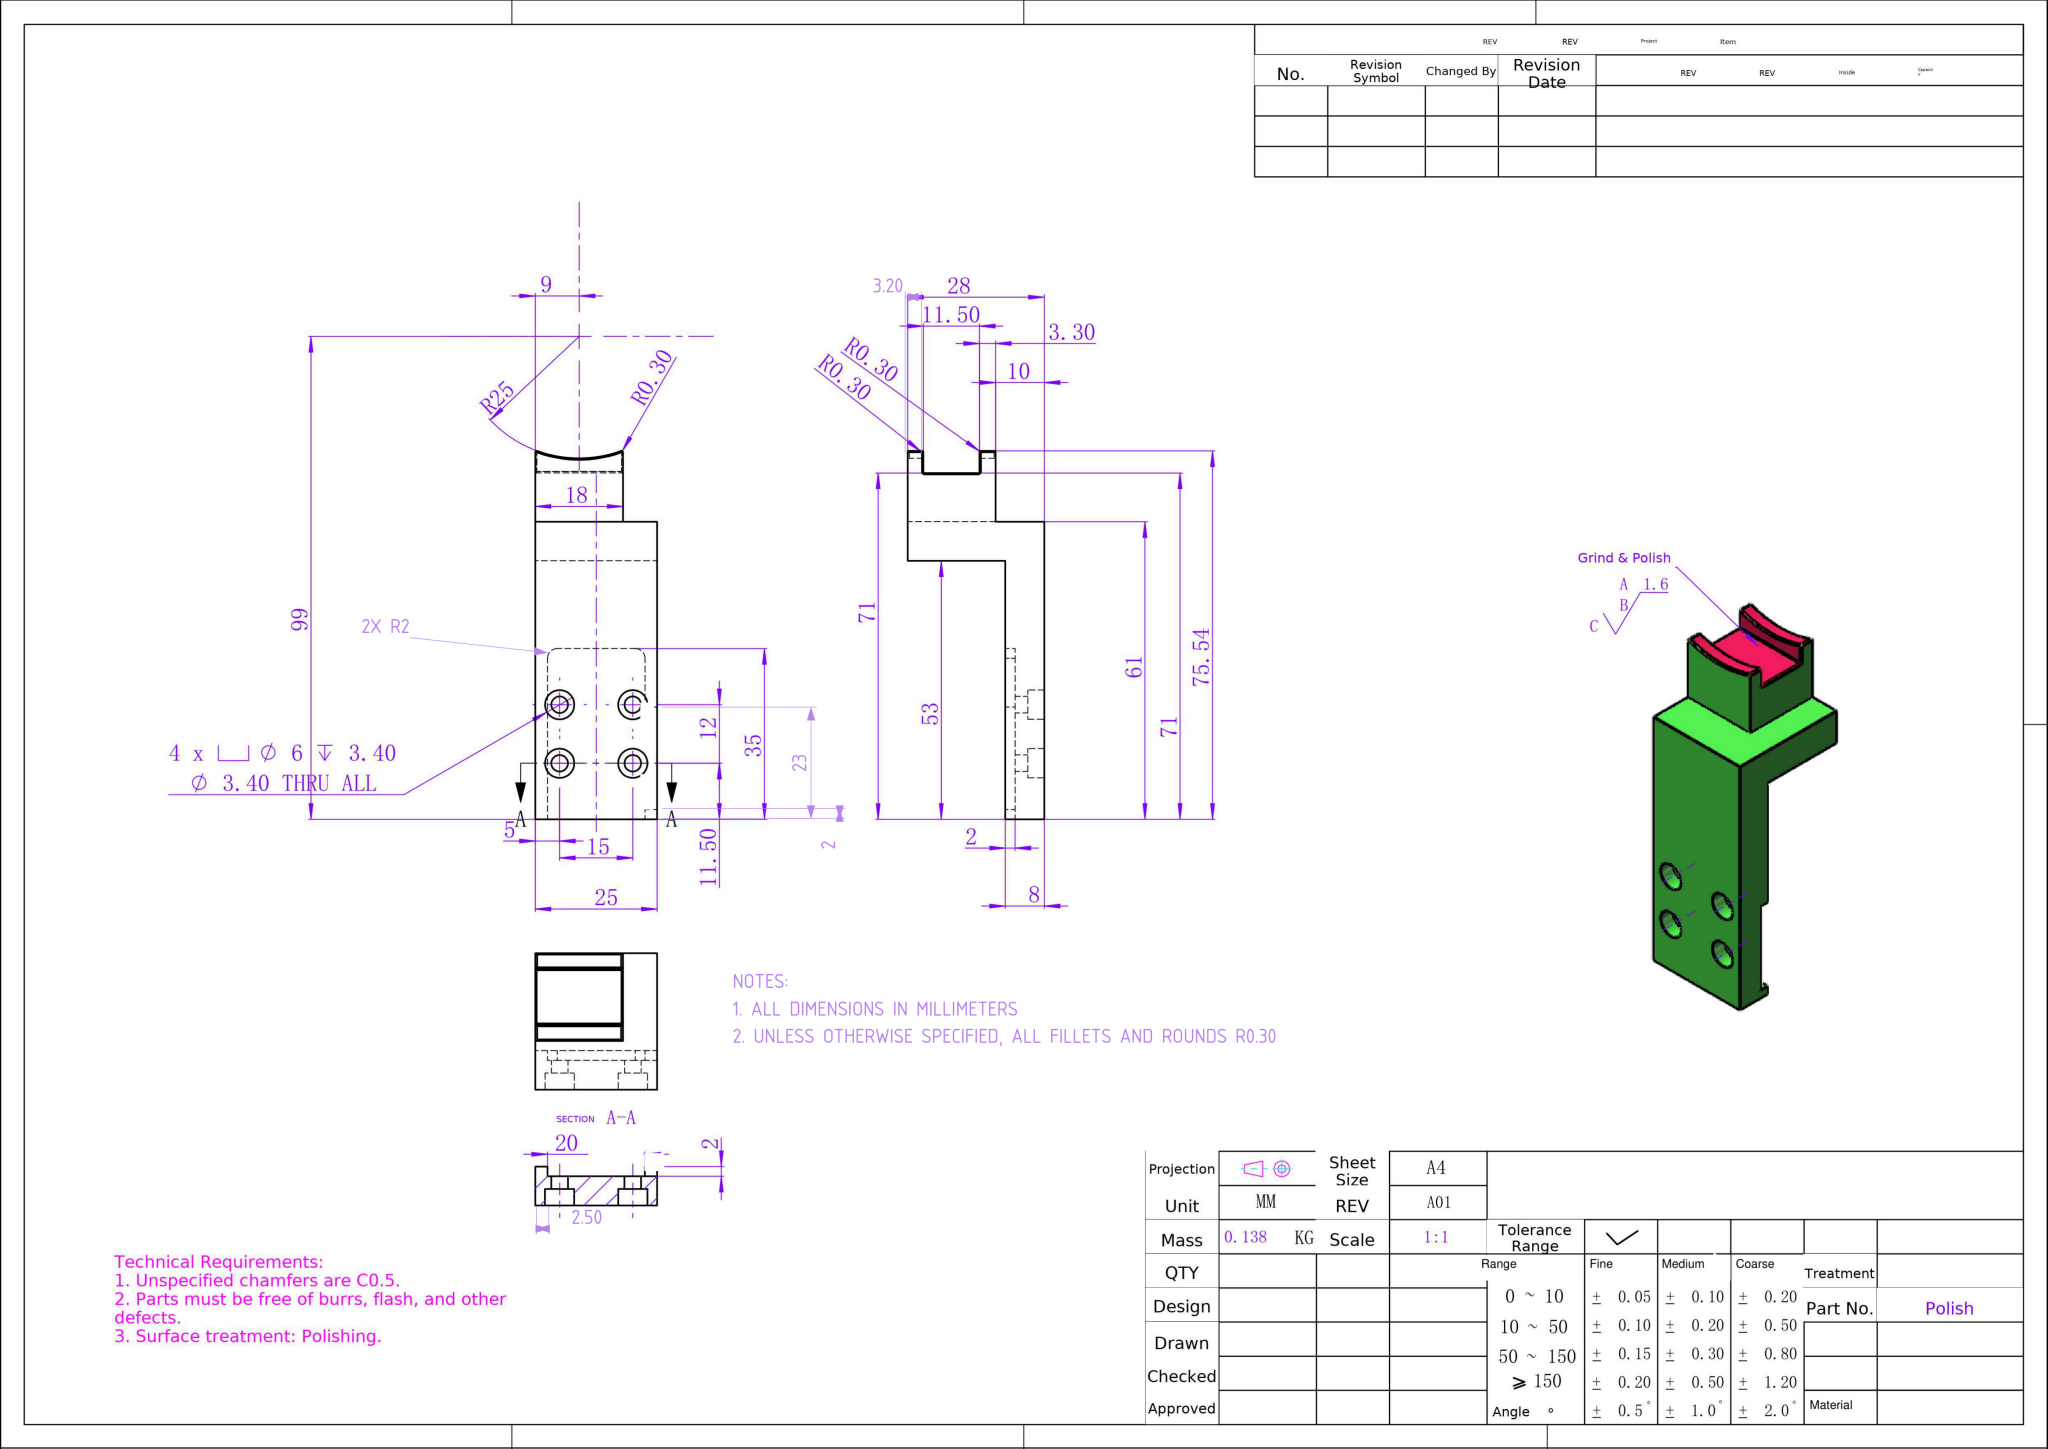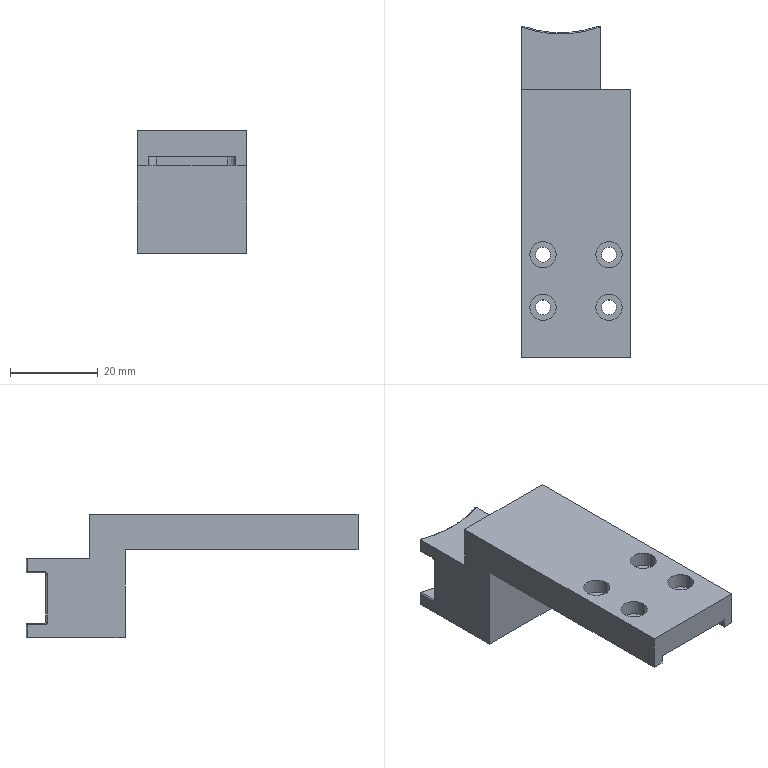Part | NX | mm | 1 solid | 69 faces | box 25 x 75.54 x 28 mm | volume 17873 mm3 | cylinder 32 | plane 25 | torus 8 | sphere 4 | commonest cylinder face diameters 0.6 x12 3.4 x8 6 x8 50 x2 4 x2